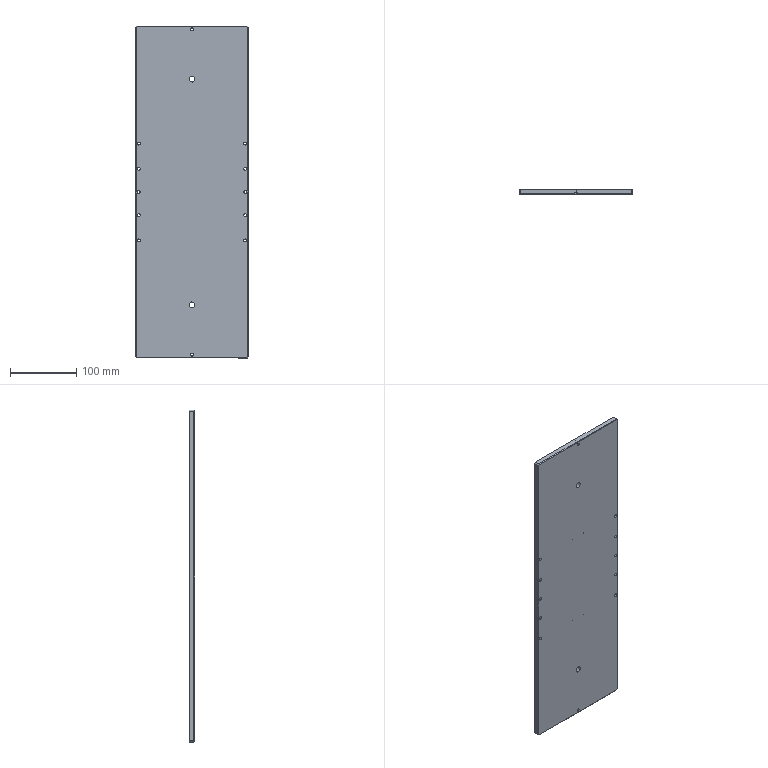Component | SolidWorks | 012-1 | 1 solid | 98 faces | box 170 x 8 x 500 mm | volume 674517 mm3 | cylinder 60 | plane 30 | cone 8 | commonest cylinder face diameters 8 x24 4.5 x24 4.2 x8 8.8 x4 | material AL6061
build123d program:
from build123d import *

# Parameters (mm, degrees)
SKETCH1_W                                         = 500
SKETCH1_H                                         = 170
BOSS_EXTRUDE1_DEPTH                               = 8
CHAMFER1_SIZE                                     = 2
G1_8_TAPPED_HOLE1_D                               = 8.8
G1_8_TAPPED_HOLE1_DEPTH                           = 22.18
G1_8_TAPPED_HOLE1_TIP                             = 2.644
HOLE_SIZE_ACCORDING_TO_TYPE_OF_HEX_SO_D           = 4.5
HOLE_SIZE_ACCORDING_TO_TYPE_OF_HEX_SO_DEPTH       = 22.18
HOLE_SIZE_ACCORDING_TO_TYPE_OF_HEX_SO_CBORE_D     = 8
HOLE_SIZE_ACCORDING_TO_TYPE_OF_HEX_SO_CBORE_DEPTH = 4.6
HOLE_SIZE_ACCORDING_TO_TYPE_OF_HEX_SO_TIP         = 1.352
CHAMFER2_SIZE                                     = 1
M5_TAPPED_HOLE1_D                                 = 4.2
M5_TAPPED_HOLE1_DEPTH                             = 6
M5_TAPPED_HOLE1_TIP                               = 1.262


with BuildPart() as part:
    # Sketch1 → Boss-Extrude1 (new body)
    with BuildSketch(Plane.XY):
        Rectangle(SKETCH1_W, SKETCH1_H)
    extrude(amount=BOSS_EXTRUDE1_DEPTH)

    # Chamfer1
    chamfer1_edges = [part.edges().sort_by_distance(p)[0] for p in [
        (250, -85, 4),
        (-250, -85, 4),
        (-250, 85, 4),
        (250, 85, 4),
    ]]
    chamfer(chamfer1_edges, length=CHAMFER1_SIZE)

    # G1_8 Tapped Hole1
    with Locations(Plane(origin=(0, 0, 0), x_dir=(-1, 0, 0), z_dir=(0, 0, -1))):
        with Locations((-170, 0), (170, 0)):
            Hole(G1_8_TAPPED_HOLE1_D / 2, depth=G1_8_TAPPED_HOLE1_DEPTH)
            with Locations((0, 0, -(G1_8_TAPPED_HOLE1_DEPTH + G1_8_TAPPED_HOLE1_TIP / 2))):  # 118° drill point
                Cone(0, G1_8_TAPPED_HOLE1_D / 2, G1_8_TAPPED_HOLE1_TIP, mode=Mode.SUBTRACT)

    # Hole Size _ according to_ type of hex so
    with Locations(Plane(origin=(0, 0, 0), x_dir=(-1, 0, 0), z_dir=(0, 0, -1))):
        with Locations((-245, 0), (245, 0), (0, 80.25), (0, -80.25), (-35, 80.25), (-73, 80.25), (-35, -80.25), (-73, -80.25), (35, 80.25), (35, -80.25), (73, -80.25), (73, 80.25)):
            CounterBoreHole(HOLE_SIZE_ACCORDING_TO_TYPE_OF_HEX_SO_D / 2, HOLE_SIZE_ACCORDING_TO_TYPE_OF_HEX_SO_CBORE_D / 2, HOLE_SIZE_ACCORDING_TO_TYPE_OF_HEX_SO_CBORE_DEPTH, depth=HOLE_SIZE_ACCORDING_TO_TYPE_OF_HEX_SO_DEPTH)
            with Locations((0, 0, -(HOLE_SIZE_ACCORDING_TO_TYPE_OF_HEX_SO_DEPTH + HOLE_SIZE_ACCORDING_TO_TYPE_OF_HEX_SO_TIP / 2))):  # 118° drill point
                Cone(0, HOLE_SIZE_ACCORDING_TO_TYPE_OF_HEX_SO_D / 2, HOLE_SIZE_ACCORDING_TO_TYPE_OF_HEX_SO_TIP, mode=Mode.SUBTRACT)

    # Chamfer2
    chamfer2_edges = [part.edges().sort_by_distance(p)[0] for p in [
        (0, -85, 8),
        (-250, 0, 8),
        (250, 0, 8),
        (0, 85, 8),
        (249, 84, 8),
        (249, -84, 8),
        (-249, 84, 8),
        (-249, -84, 8),
    ]]
    chamfer(chamfer2_edges, length=CHAMFER2_SIZE)

    # M5 Tapped Hole1
    with Locations(Plane(origin=(0, 0, 0), x_dir=(-1, 0, 0), z_dir=(0, 0, -1))):
        with Locations((-75, 11.5), (75, 11.5), (75, -11.5), (-75, -11.5)):
            Hole(M5_TAPPED_HOLE1_D / 2, depth=M5_TAPPED_HOLE1_DEPTH)
            with Locations((0, 0, -(M5_TAPPED_HOLE1_DEPTH + M5_TAPPED_HOLE1_TIP / 2))):  # 118° drill point
                Cone(0, M5_TAPPED_HOLE1_D / 2, M5_TAPPED_HOLE1_TIP, mode=Mode.SUBTRACT)


solid = part.part

# Placed as in the assembly
solid = solid.moved(Location((-240.455, -163.942, -258.376), (90, 0, 90)))